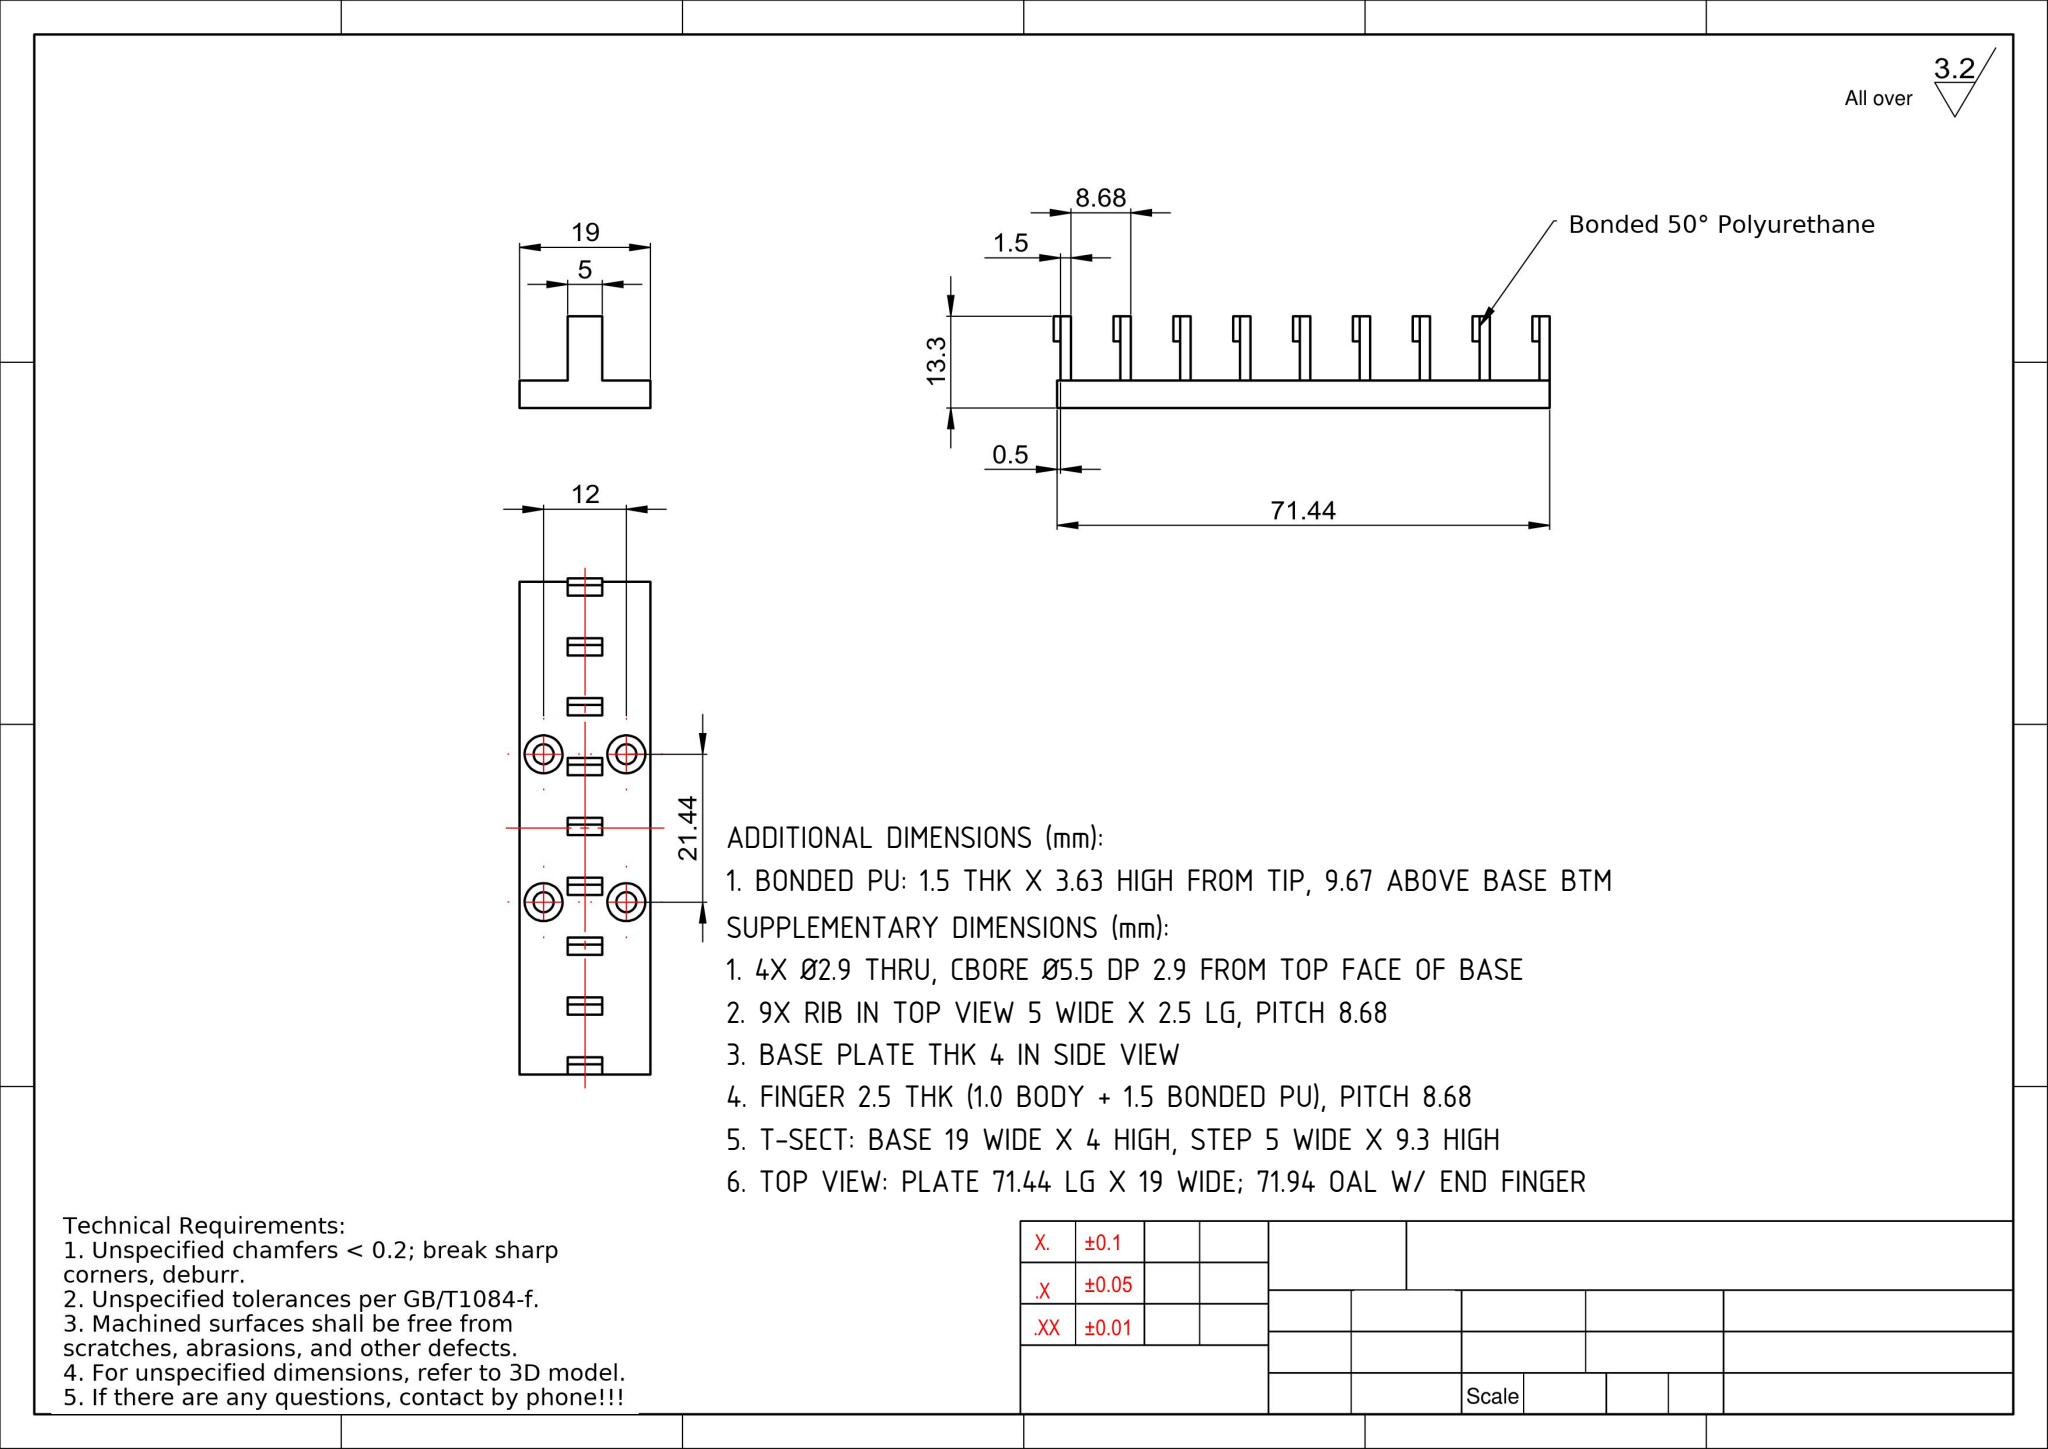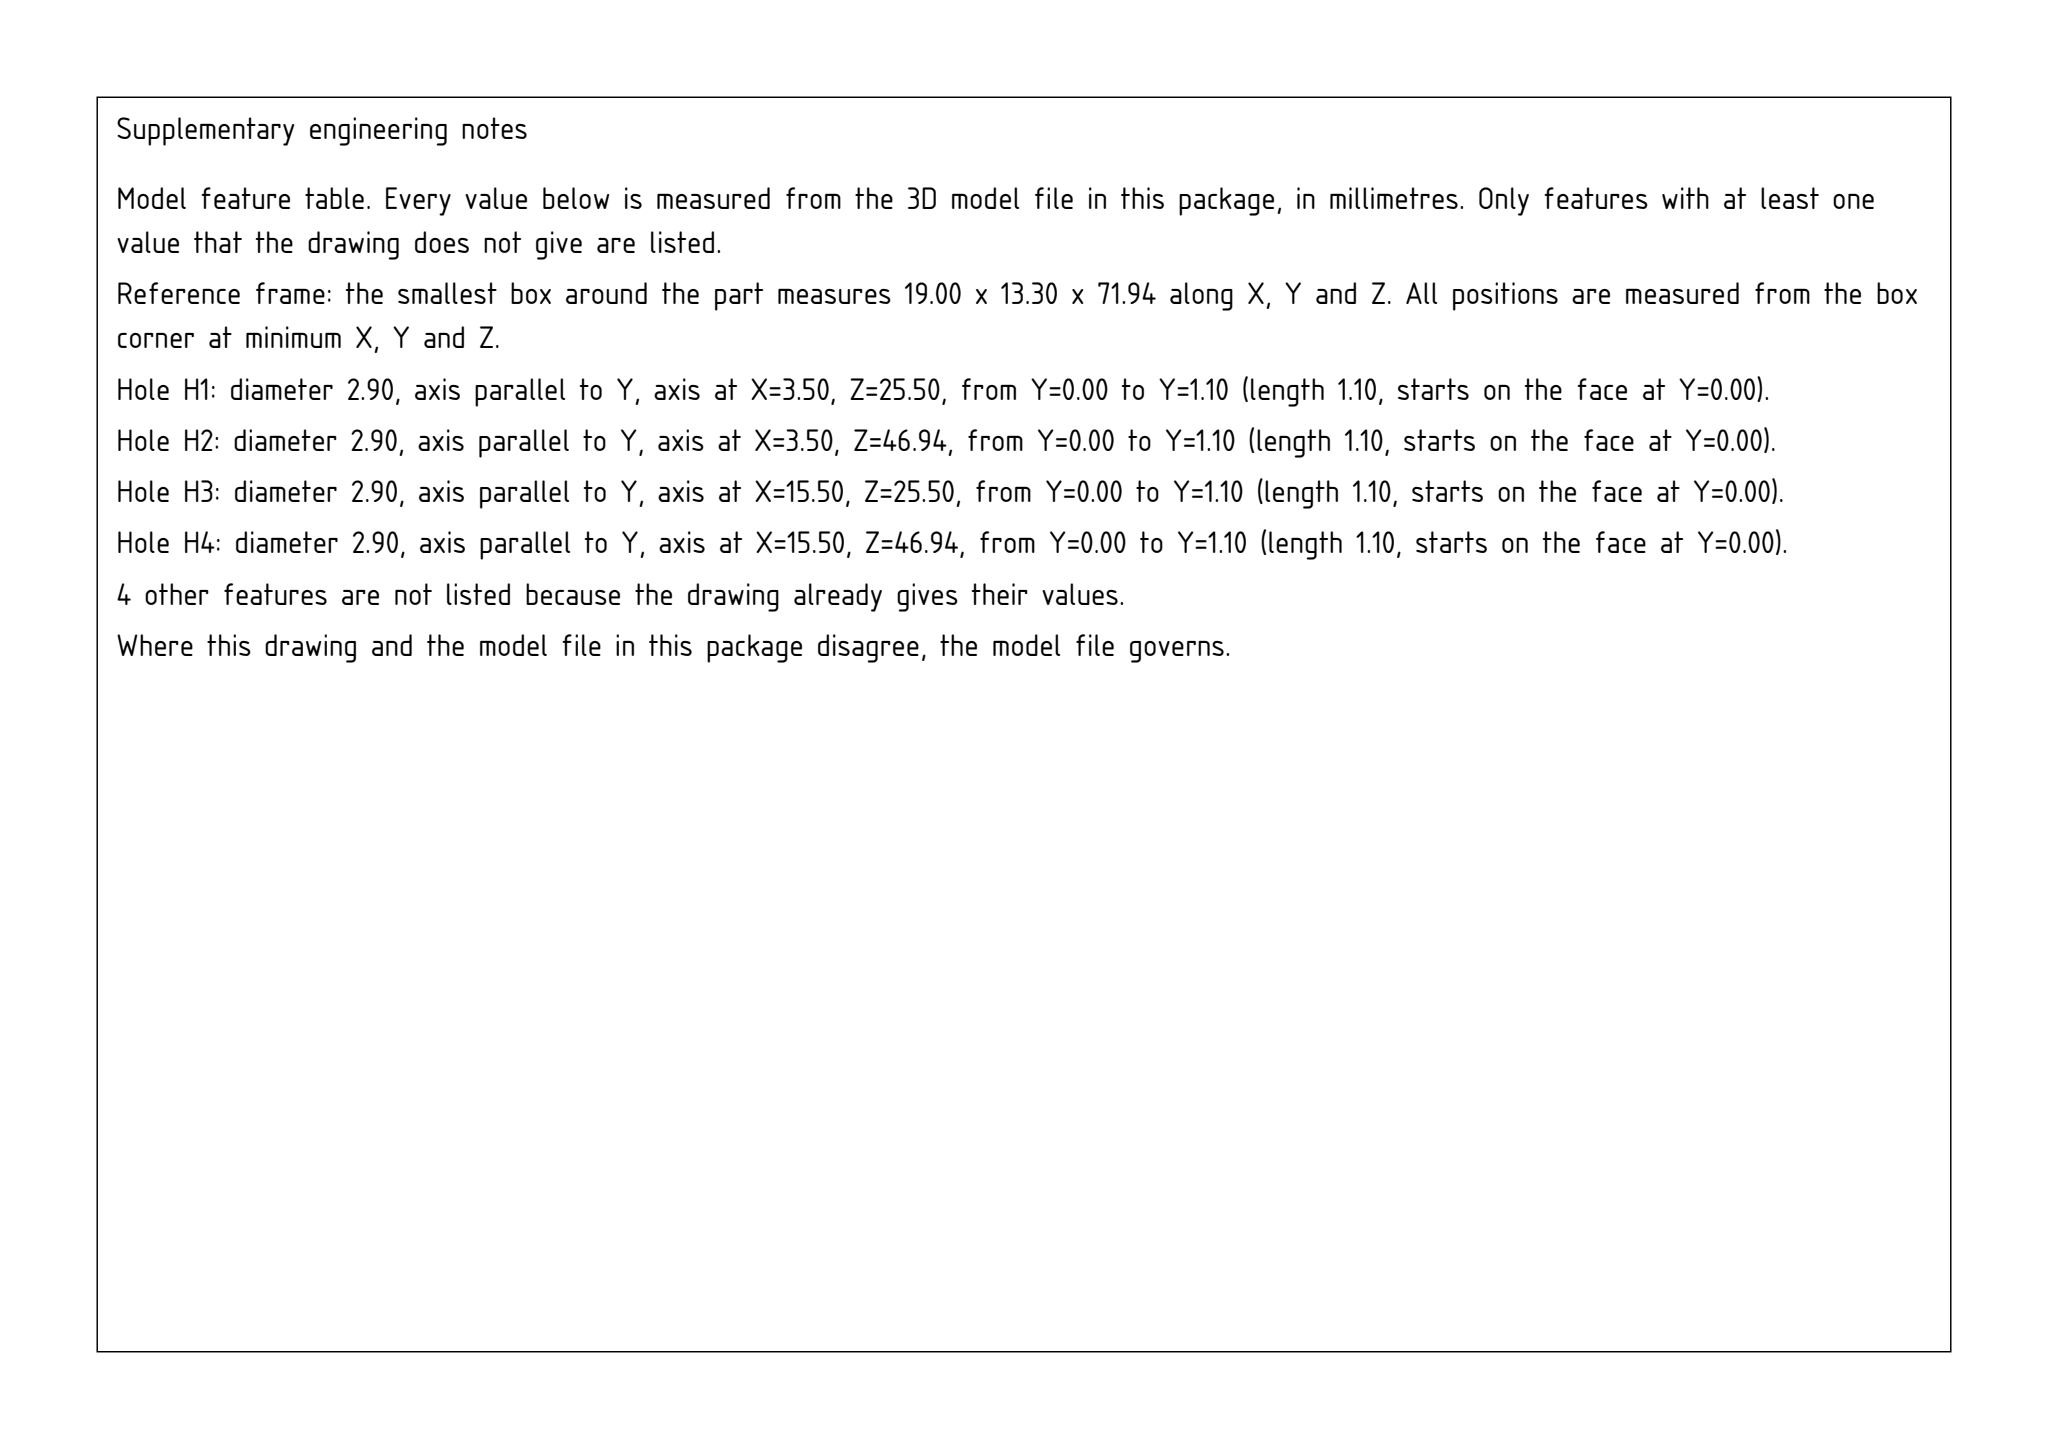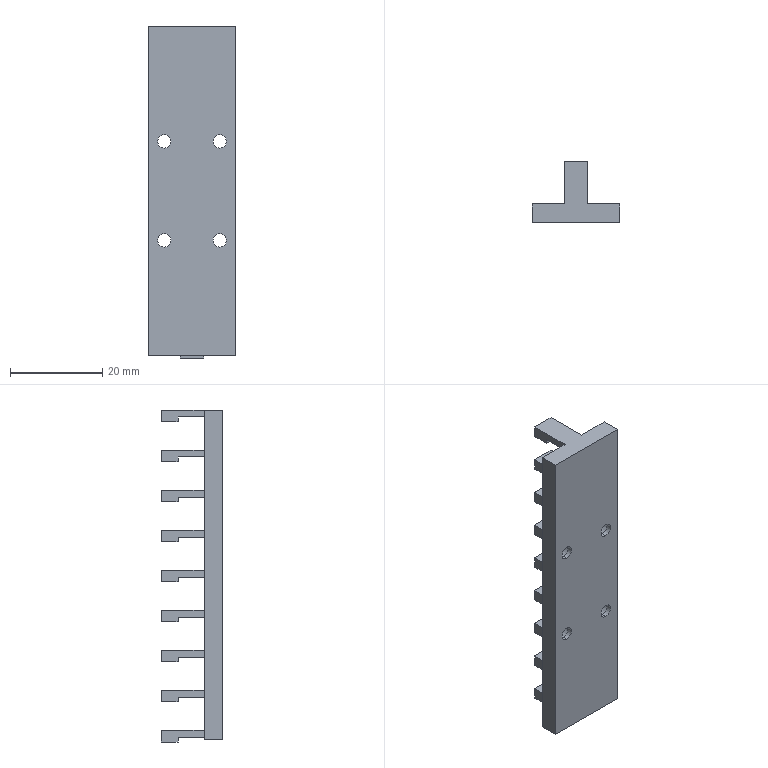Part | SolidWorks | mm | 1 solid | 88 faces | box 19 x 13.3 x 71.94 mm | volume 5916 mm3 | plane 72 | cylinder 16 | commonest cylinder face diameters 5.5 x8 2.9 x8
build123d program:
from build123d import *

# Parameters (mm, degrees)
SKETCH1_W                                         = 19
SKETCH1_H                                         = 4
BOSS_EXTRUDE1_DEPTH                               = 35.72
SKETCH2_W                                         = 5
SKETCH2_H                                         = 1.5
BOSS_EXTRUDE2_DEPTH                               = 9.3
LPATTERN1_COUNT                                   = 9
LPATTERN1_PITCH                                   = 8.68
M2_5_HEX_SOCKET_HEAD_CAP_SCREW_CBORE1_D           = 2.9
M2_5_HEX_SOCKET_HEAD_CAP_SCREW_CBORE1_CBORE_D     = 5.5
M2_5_HEX_SOCKET_HEAD_CAP_SCREW_CBORE1_CBORE_DEPTH = 2.9
SKETCH5_W                                         = 5
SKETCH5_H                                         = 3.628
BOSS_EXTRUDE3_DEPTH                               = 1
LPATTERN2_COUNT                                   = 9
LPATTERN2_PITCH                                   = 8.68


with BuildPart() as part:
    # Sketch1 → Boss-Extrude1 (new, symmetric)
    with BuildSketch(Plane.XY):
        Rectangle(SKETCH1_W, SKETCH1_H)
    extrude(amount=BOSS_EXTRUDE1_DEPTH, both=True)

    # Sketch2 → Boss-Extrude2 (add)
    with BuildSketch(Plane(origin=(0, 2, 0), x_dir=(1, 0, 0), z_dir=(0, 1, 0))):
        with Locations((0, -34.97)):
            Rectangle(SKETCH2_W, SKETCH2_H)
    boss_extrude2 = extrude(amount=BOSS_EXTRUDE2_DEPTH)

    # LPattern1: Boss-Extrude2 ×9
    with Locations(*[(0, 0, -i * LPATTERN1_PITCH) for i in range(1, LPATTERN1_COUNT)]):
        add(boss_extrude2)

    # M2.5 Hex Socket Head Cap Screw CBORE1 (through all)
    with Locations(Plane(origin=(0, 2, 0), x_dir=(1, 0, 0), z_dir=(0, 1, 0))):
        with Locations((-6, -10.72), (6, -10.72), (6, 10.72), (-6, 10.72)):
            CounterBoreHole(M2_5_HEX_SOCKET_HEAD_CAP_SCREW_CBORE1_D / 2, M2_5_HEX_SOCKET_HEAD_CAP_SCREW_CBORE1_CBORE_D / 2, M2_5_HEX_SOCKET_HEAD_CAP_SCREW_CBORE1_CBORE_DEPTH)


with BuildPart() as body_2:
    # Sketch5 → Boss-Extrude3 (new body)
    with BuildSketch(Plane(origin=(0, 0, 34.22), x_dir=(-1, 0, 0), z_dir=(0, 0, -1))):
        with Locations((0, 9.486)):
            Rectangle(SKETCH5_W, SKETCH5_H)
    boss_extrude3 = extrude(amount=BOSS_EXTRUDE3_DEPTH)


with BuildPart() as lpattern2_1:
    # LPattern2: pattern copy
    add(boss_extrude3.moved(Location(Vector(0, 0, -1) * (1 * LPATTERN2_PITCH))))


with BuildPart() as lpattern2_2:
    # LPattern2: pattern copy
    add(boss_extrude3.moved(Location(Vector(0, 0, -1) * (2 * LPATTERN2_PITCH))))


with BuildPart() as lpattern2_3:
    # LPattern2: pattern copy
    add(boss_extrude3.moved(Location(Vector(0, 0, -1) * (3 * LPATTERN2_PITCH))))


with BuildPart() as lpattern2_4:
    # LPattern2: pattern copy
    add(boss_extrude3.moved(Location(Vector(0, 0, -1) * (4 * LPATTERN2_PITCH))))


with BuildPart() as lpattern2_5:
    # LPattern2: pattern copy
    add(boss_extrude3.moved(Location(Vector(0, 0, -1) * (5 * LPATTERN2_PITCH))))


with BuildPart() as lpattern2_6:
    # LPattern2: pattern copy
    add(boss_extrude3.moved(Location(Vector(0, 0, -1) * (6 * LPATTERN2_PITCH))))


with BuildPart() as lpattern2_7:
    # LPattern2: pattern copy
    add(boss_extrude3.moved(Location(Vector(0, 0, -1) * (7 * LPATTERN2_PITCH))))


with BuildPart() as lpattern2_8:
    # LPattern2: pattern copy
    add(boss_extrude3.moved(Location(Vector(0, 0, -1) * (8 * LPATTERN2_PITCH))))


with BuildPart() as lpattern2_5_1:
    add(lpattern2_5.part)

    # Combine-RayDong-Repair: union body 2, LPattern2_3, LPattern2_6, LPattern2_1, LPattern2_4, LPattern2_8, part, LPattern2_7, LPattern2_2
    add(body_2.part)
    add(lpattern2_3.part)
    add(lpattern2_6.part)
    add(lpattern2_1.part)
    add(lpattern2_4.part)
    add(lpattern2_8.part)
    add(part.part)
    add(lpattern2_7.part)
    add(lpattern2_2.part)


solid = lpattern2_5_1.part